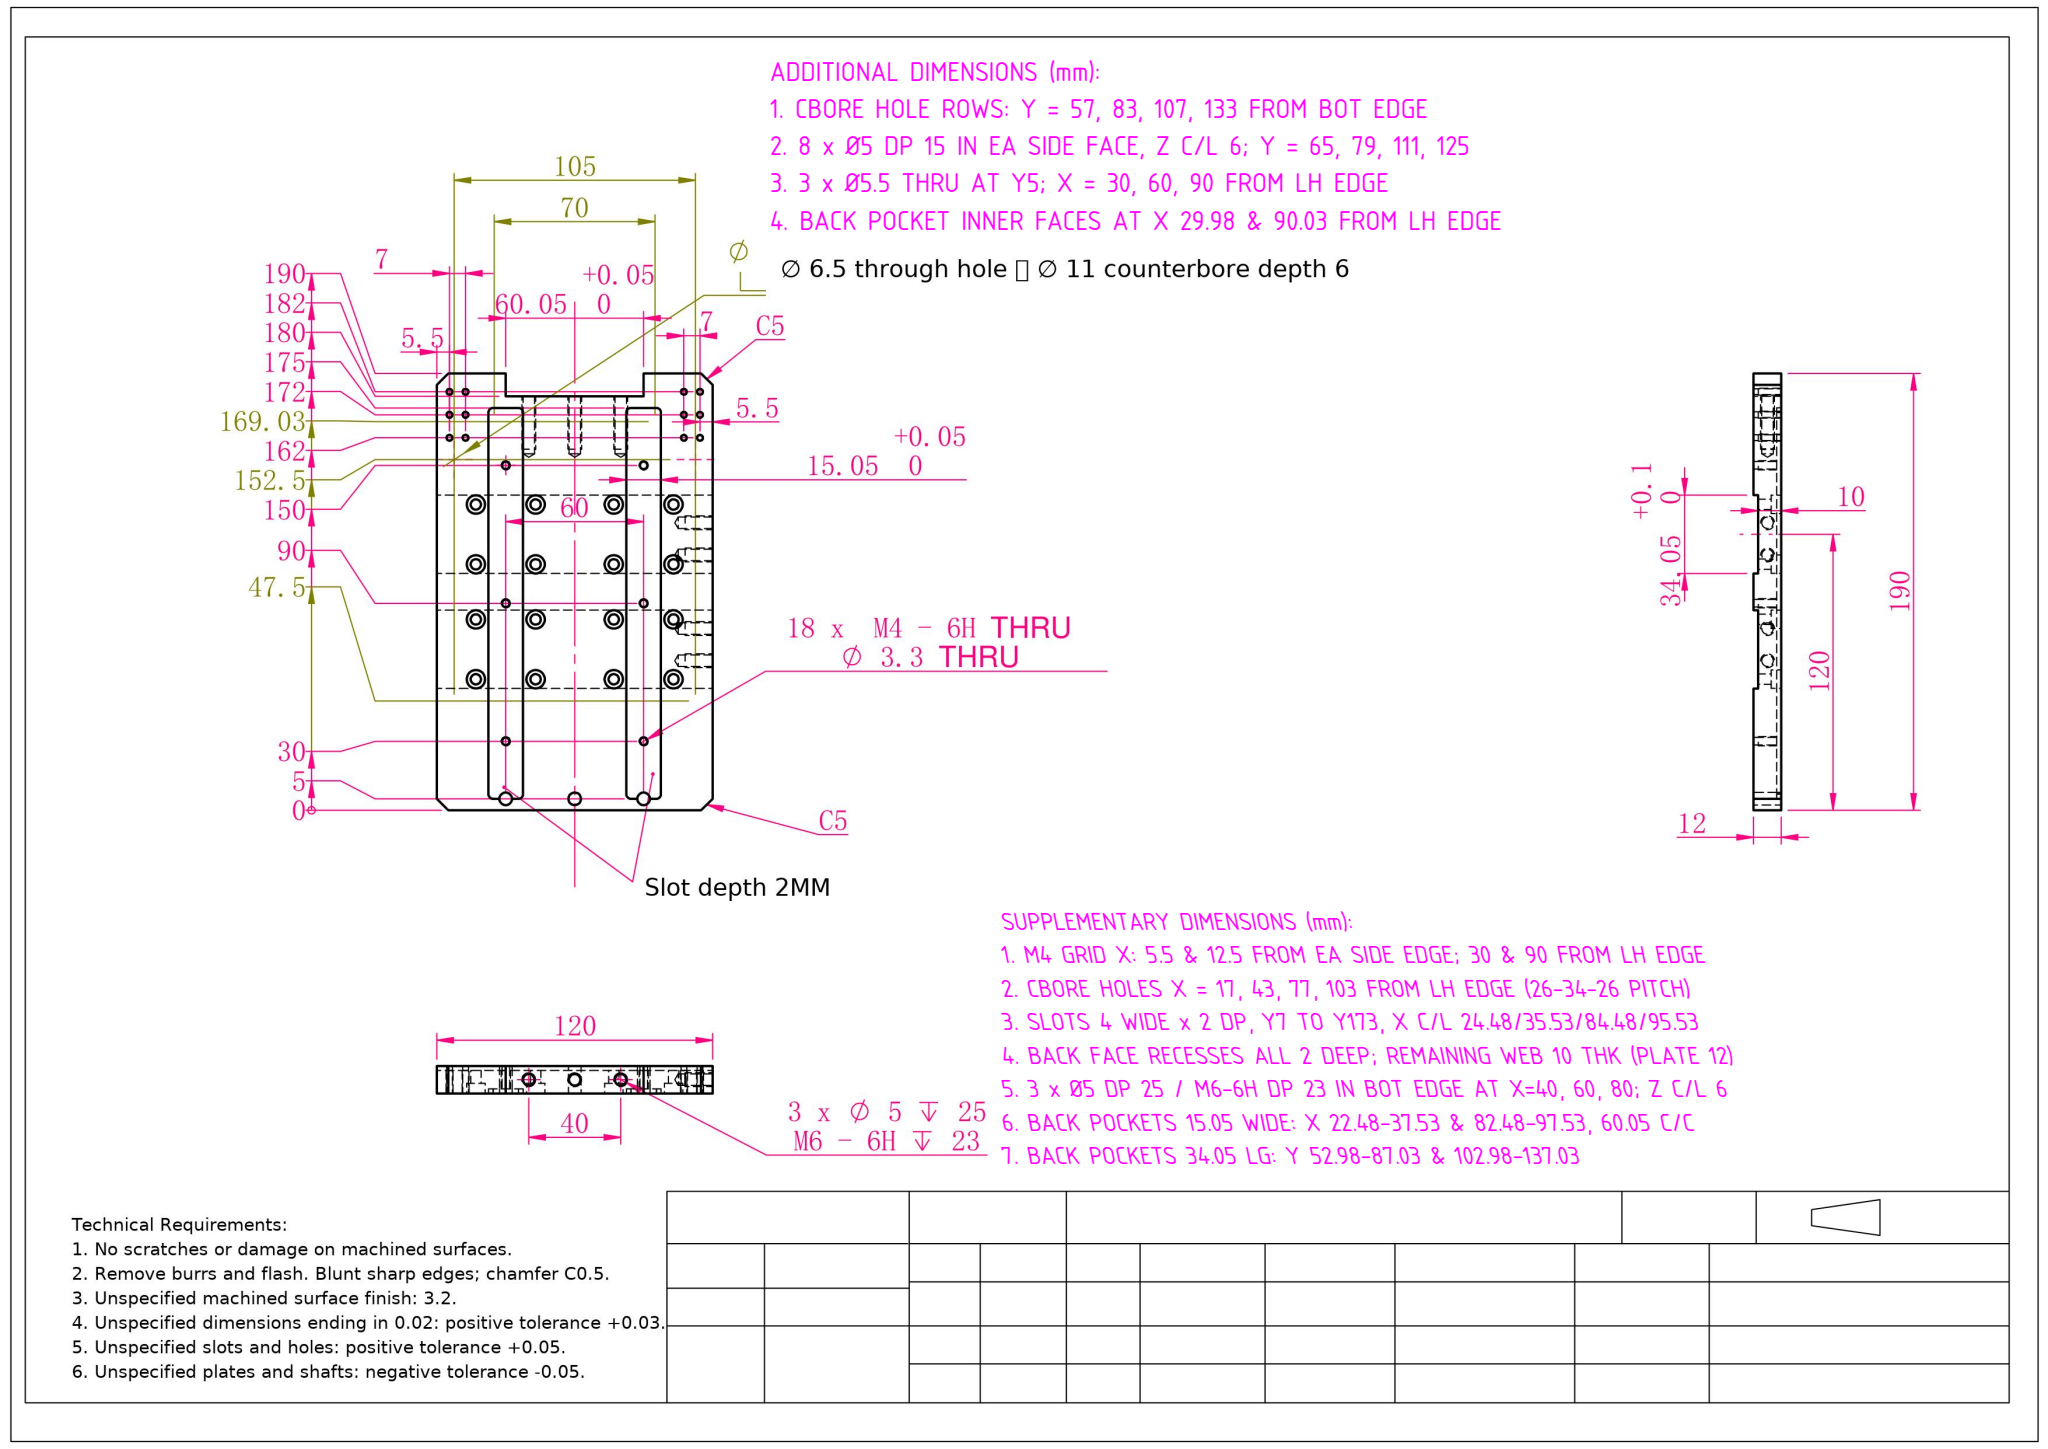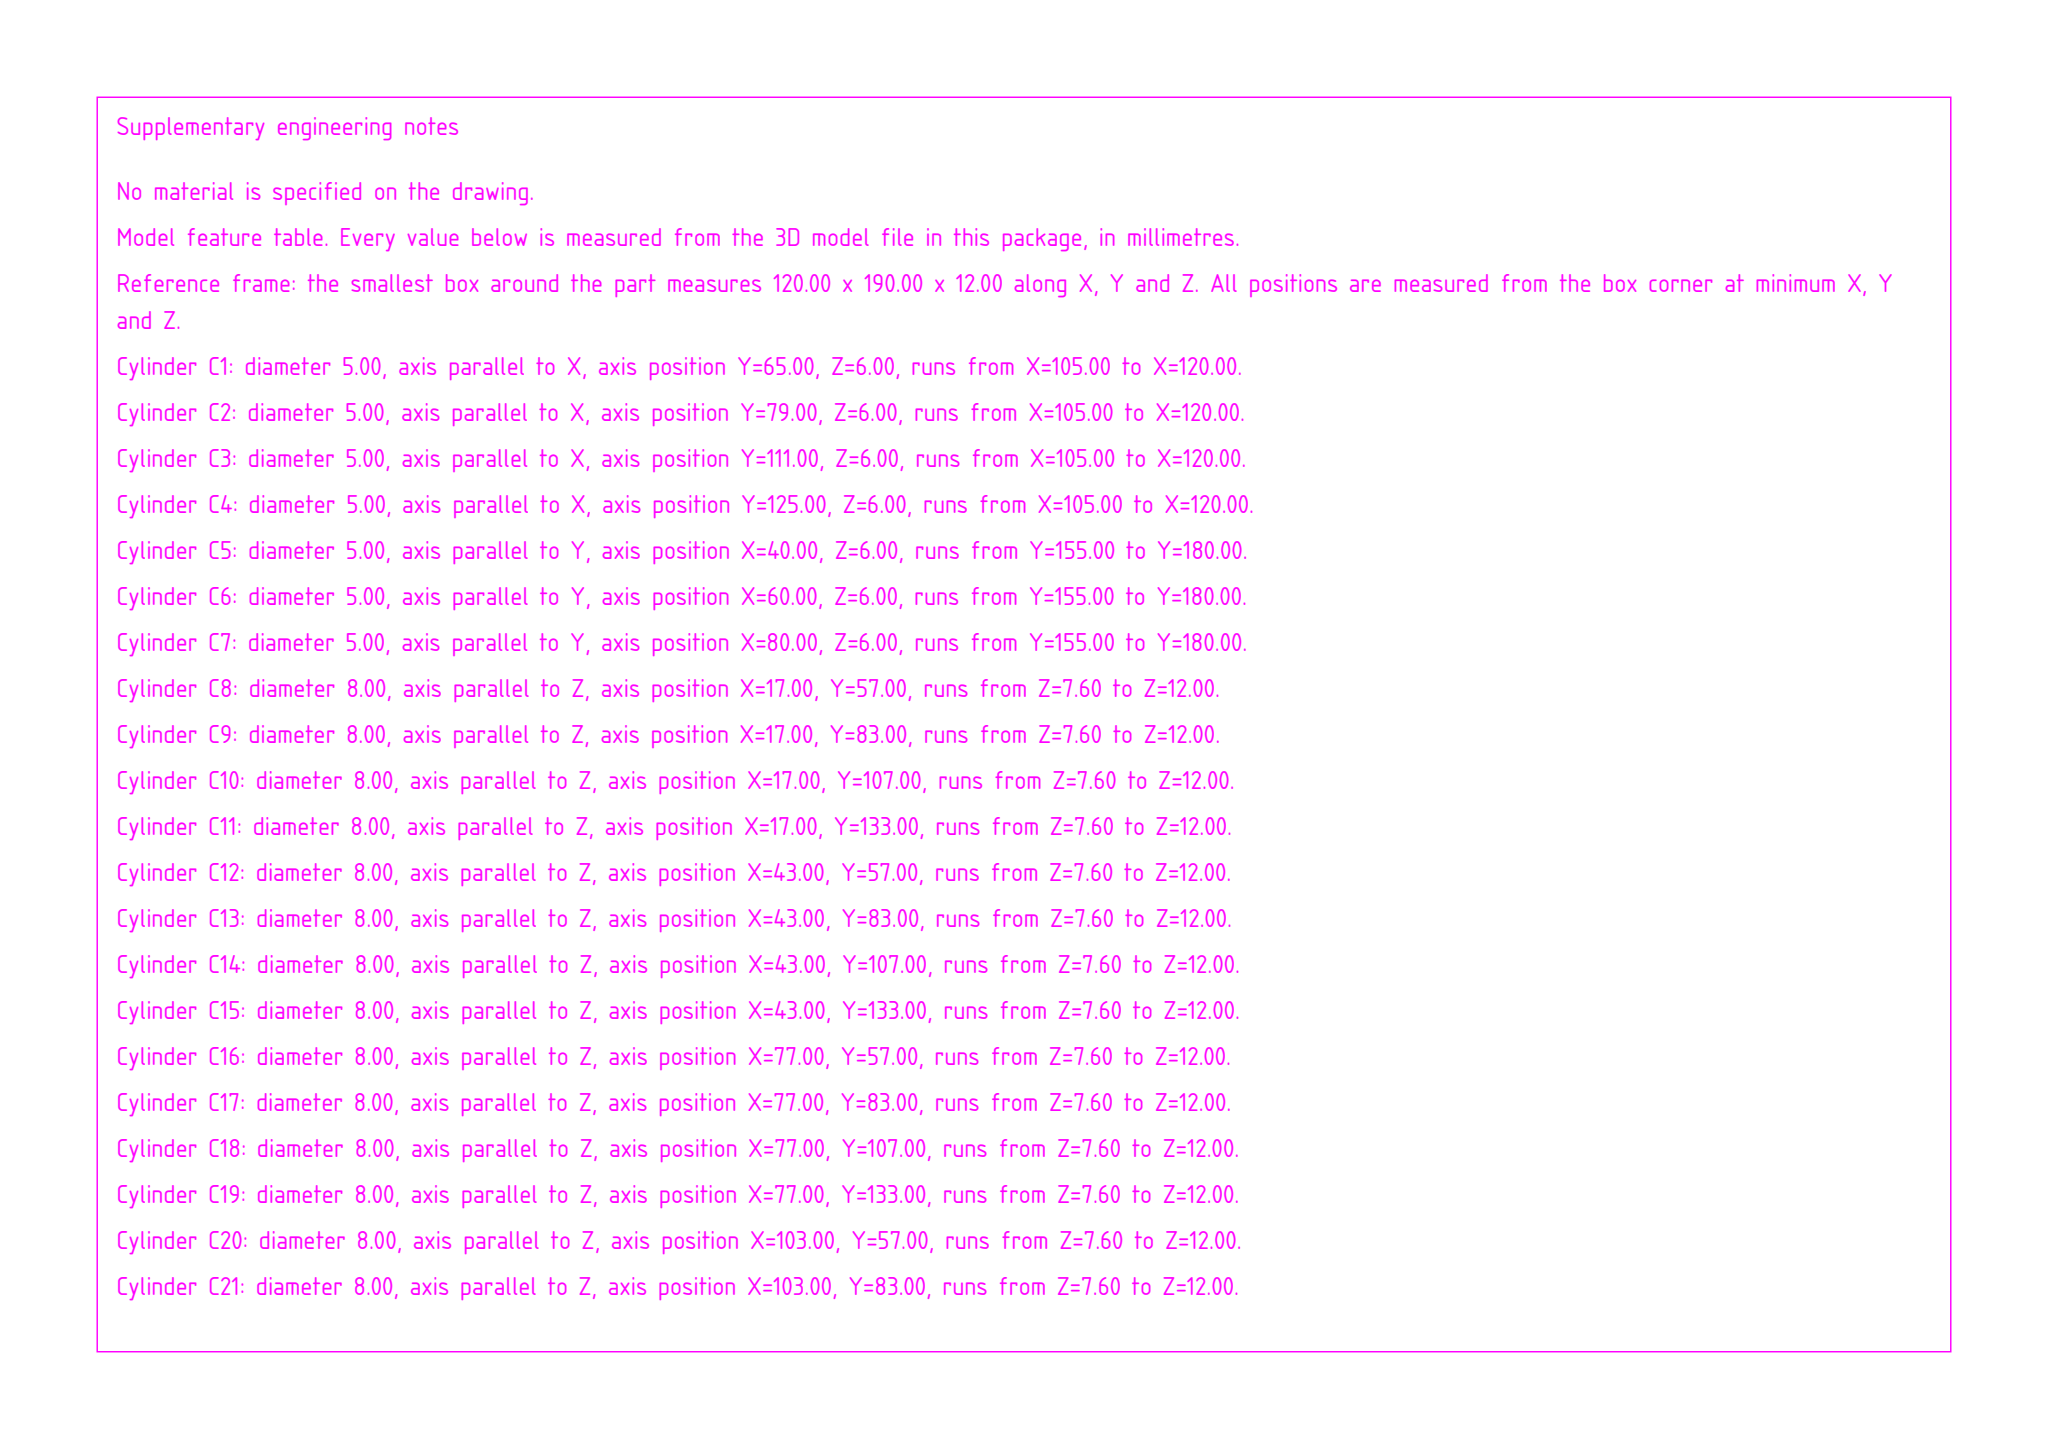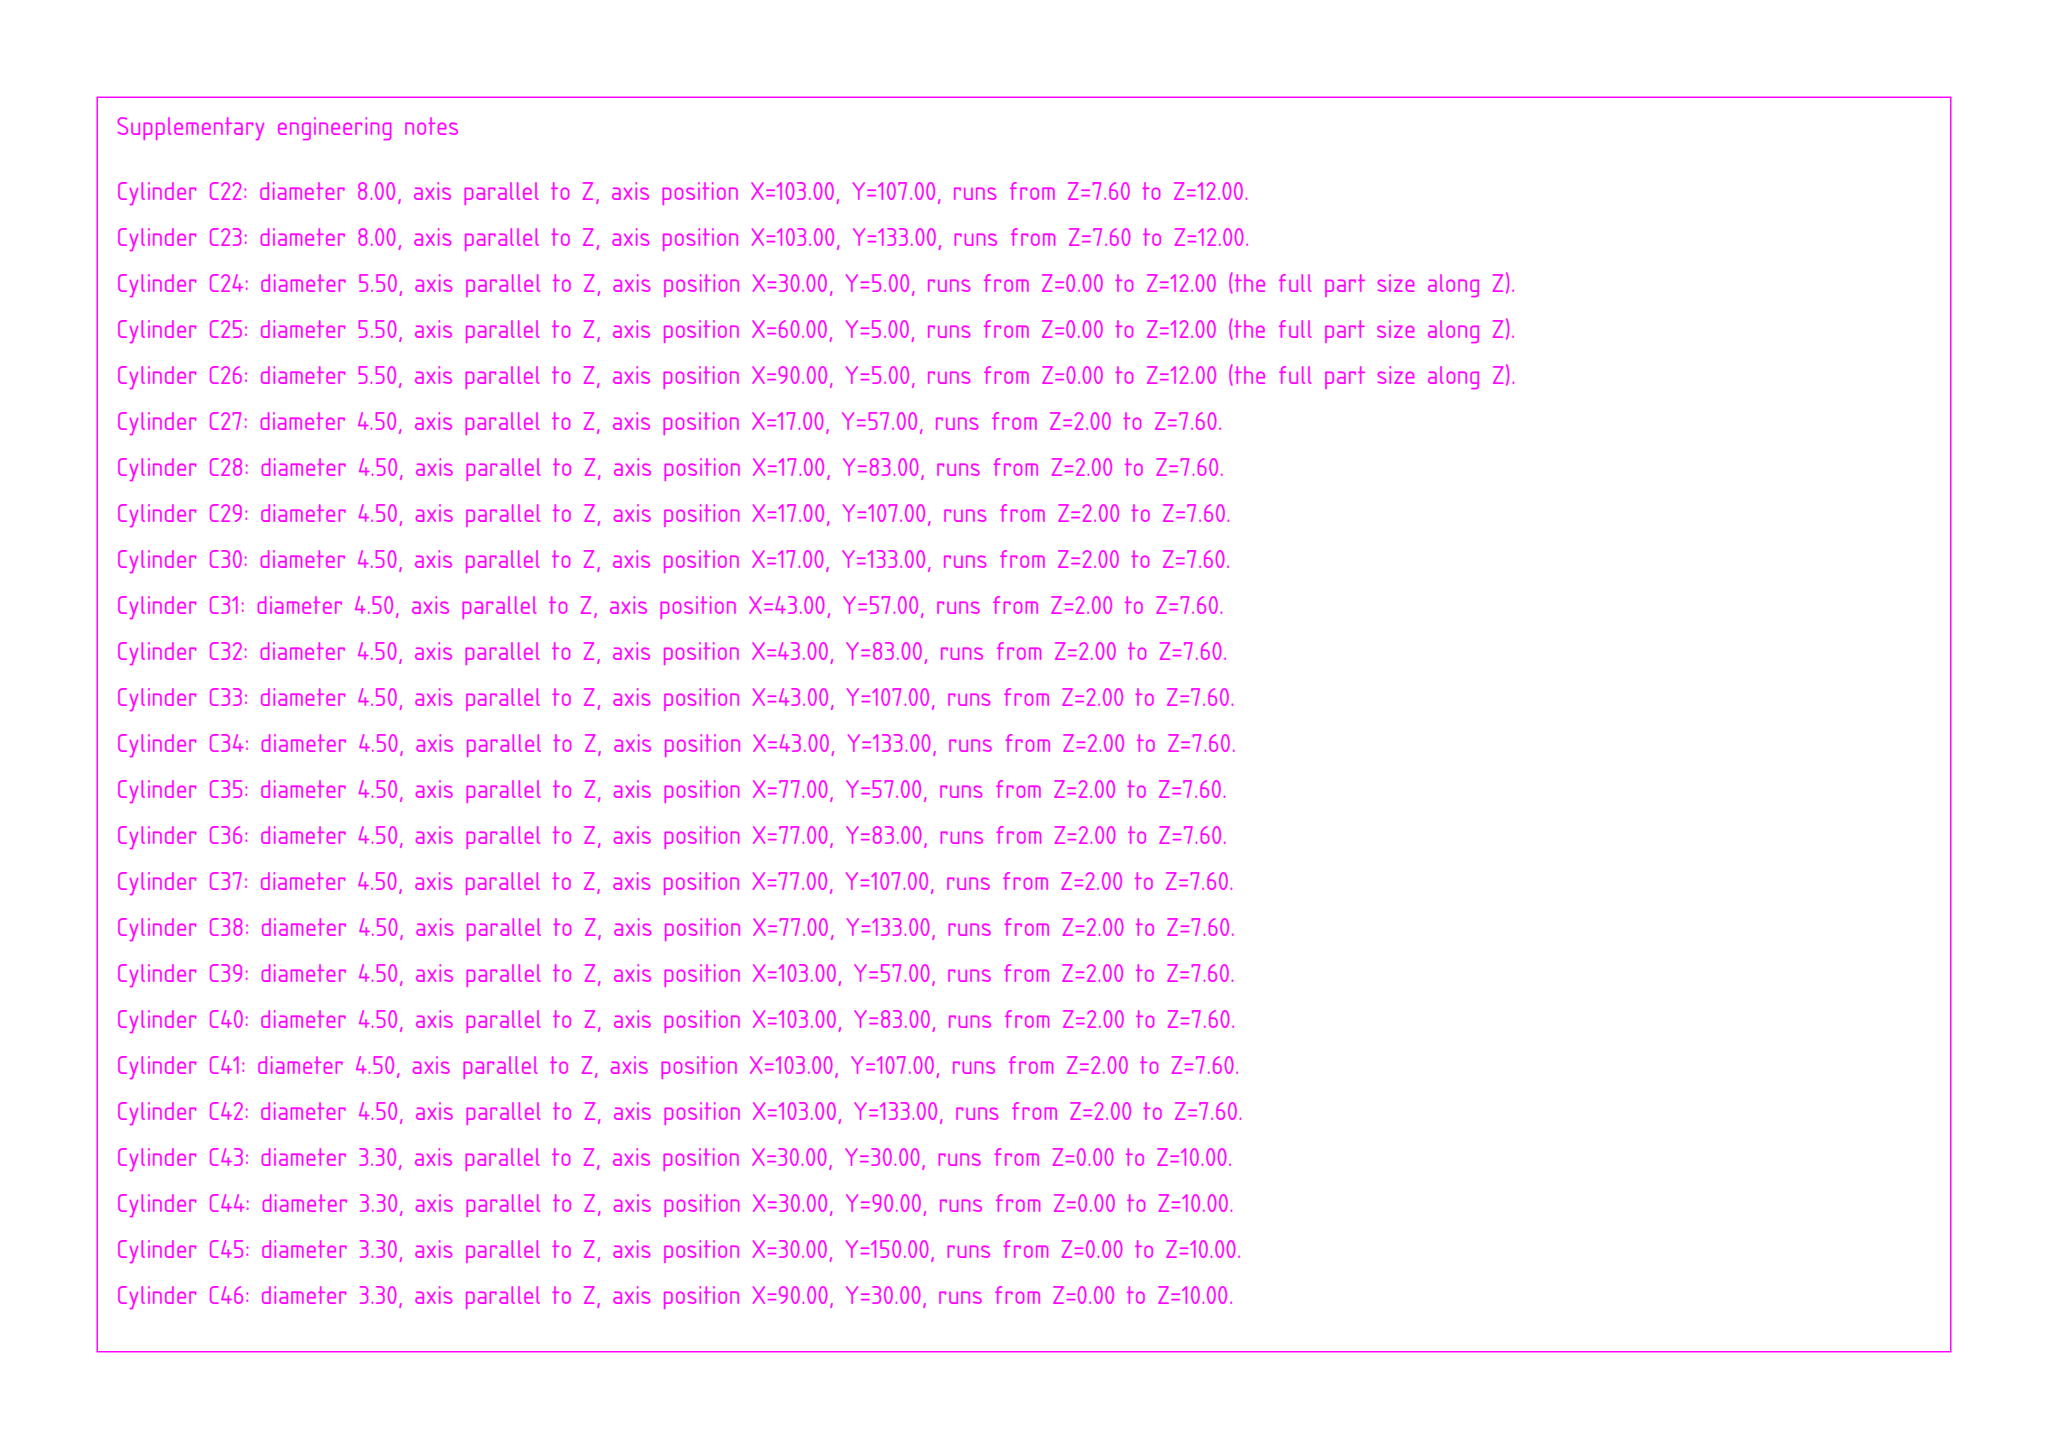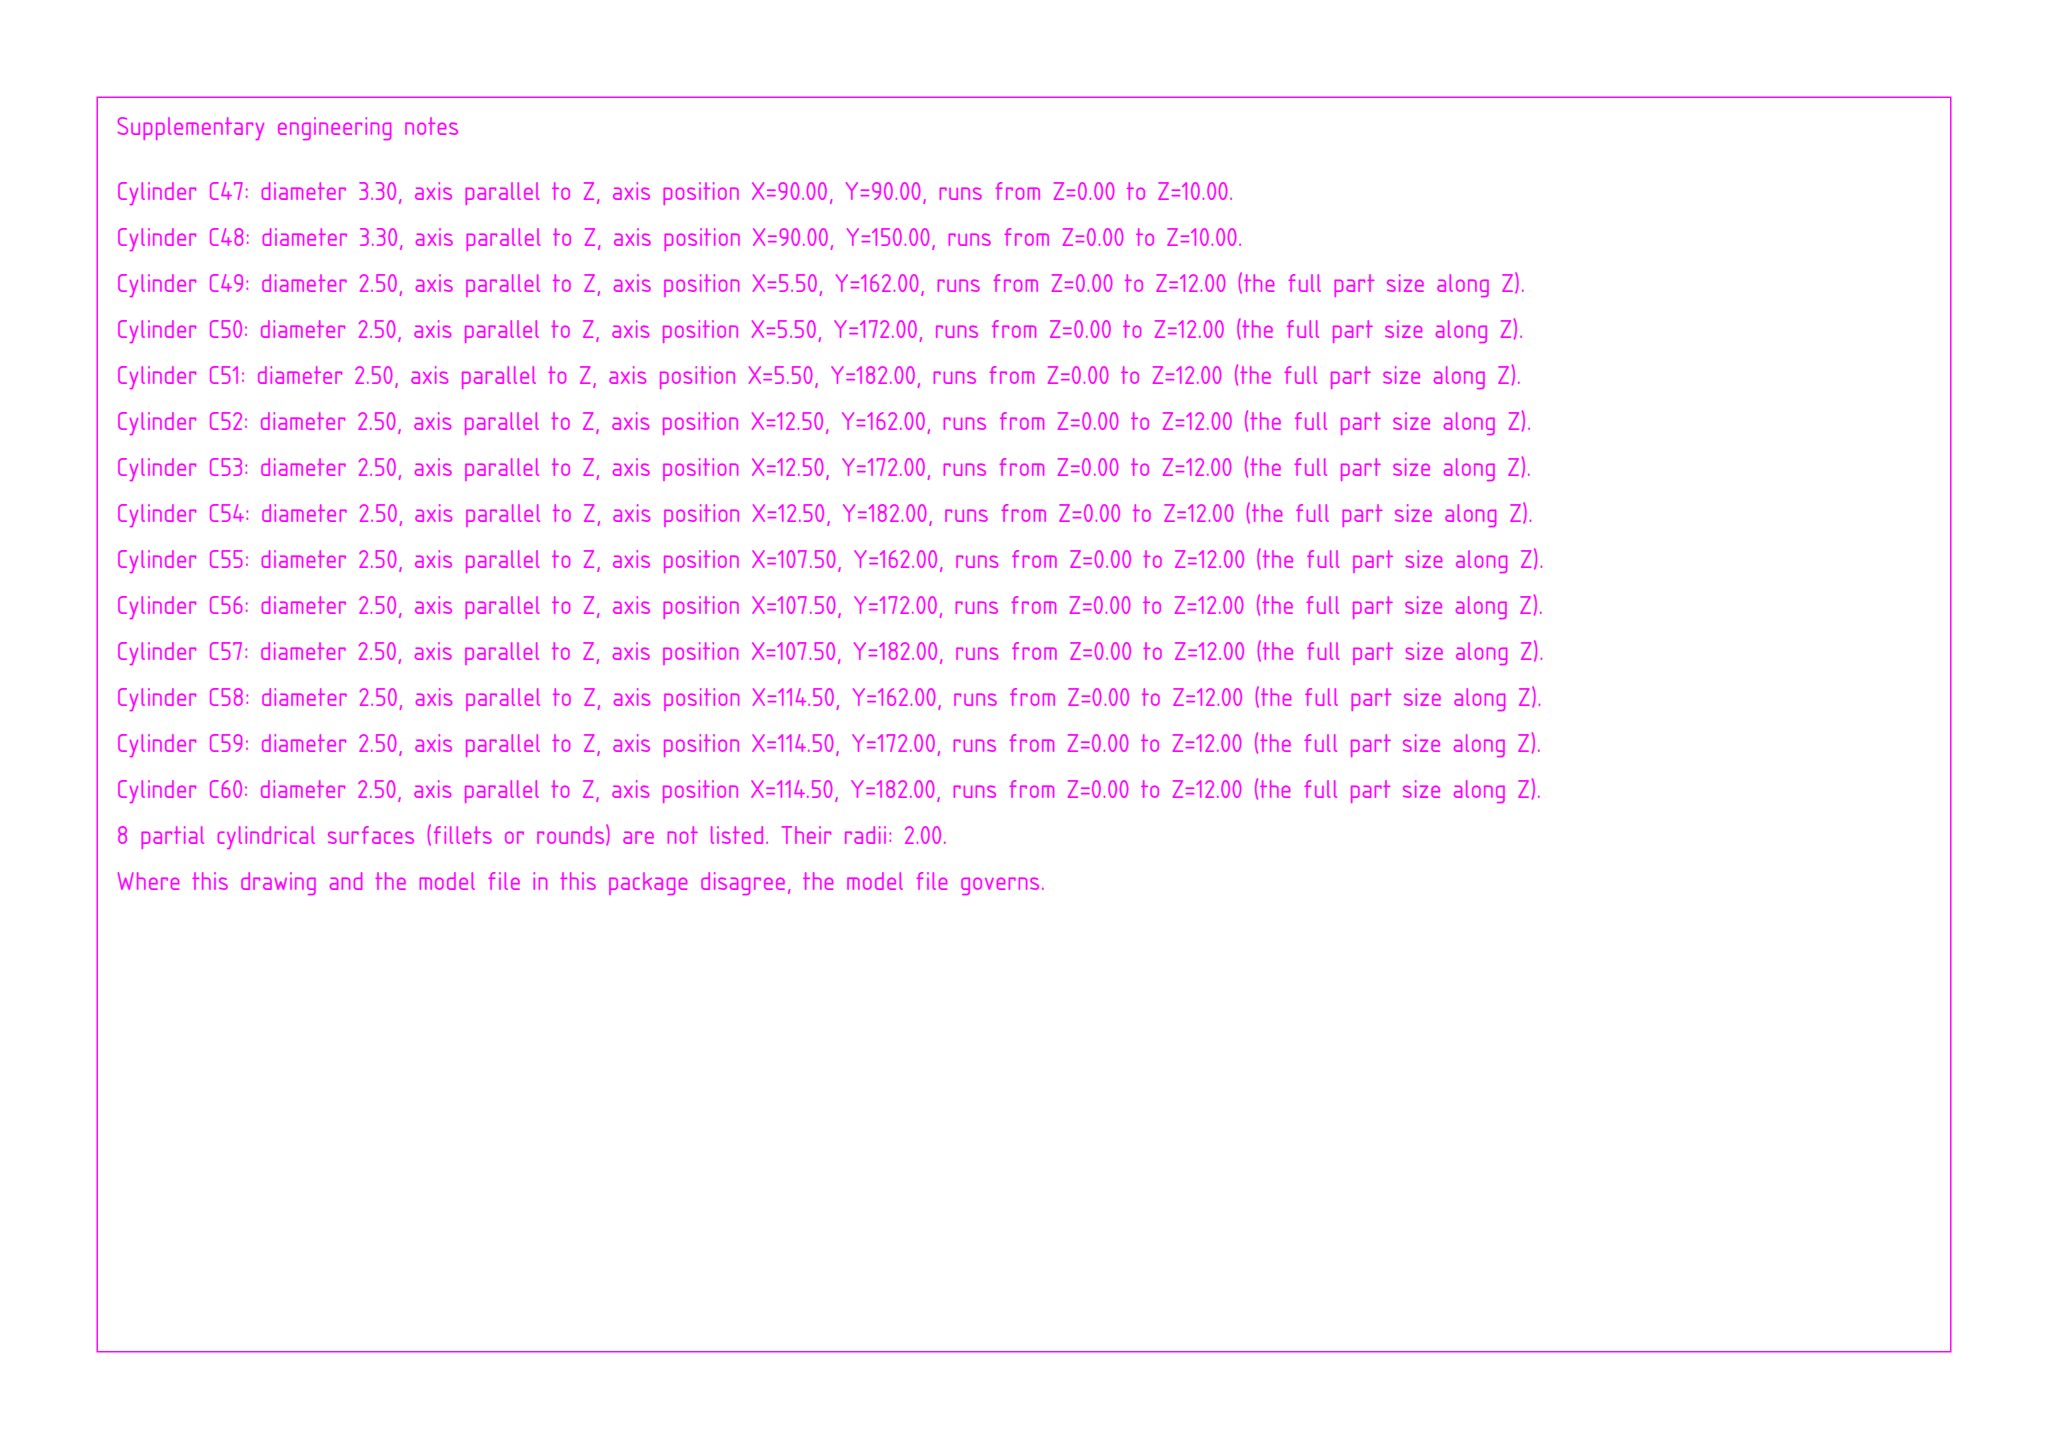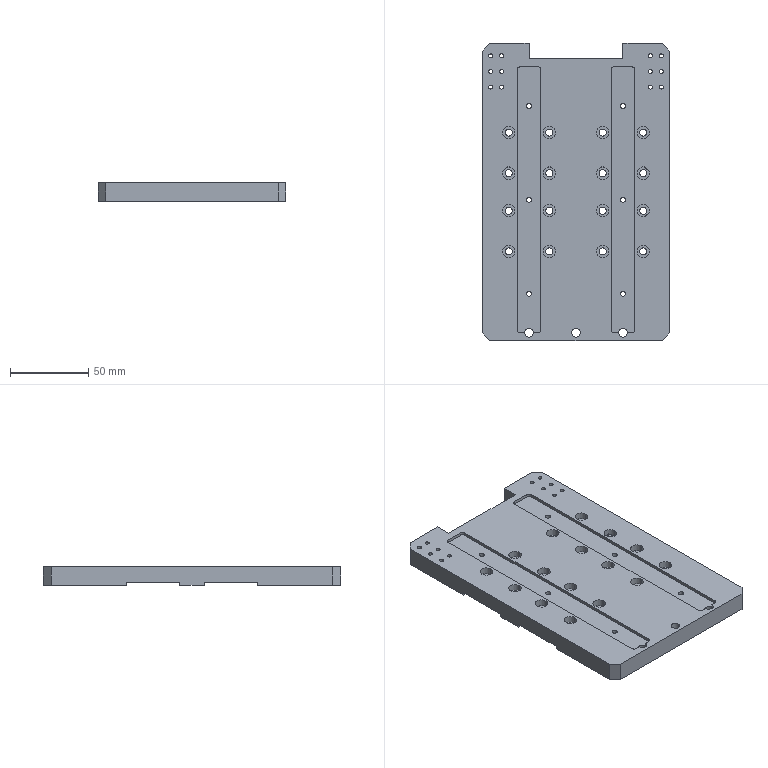Part | SolidWorks | mm | 1 solid | 192 faces | box 120 x 190 x 12 mm | volume 229520 mm3 | cylinder 128 | plane 50 | cone 14 | commonest cylinder face diameters 8 x32 4.5 x32 2.5 x24 5 x14 3.3 x12 4 x8 5.5 x6
build123d program:
from build123d import *

# Parameters (mm, degrees)
SKETCH1_W                                       = 120
SKETCH1_H                                       = 190
BOSS_EXTRUDE1_DEPTH                             = 12
M4_TAPPED_HOLE1_D                               = 3.3
SKETCH13_W                                      = 15.05
SKETCH13_H                                      = 170
CUT_EXTRUDE1_DEPTH                              = 2
SKETCH14_W                                      = 60.05
SKETCH14_H                                      = 10
CUT_EXTRUDE2_DEPTH                              = 114
M6_TAPPED_HOLE1_D                               = 5
M6_TAPPED_HOLE1_DEPTH                           = 25
M6_TAPPED_HOLE1_TIP                             = 1.502
FILLET1_R                                       = 2
M5_CLEARANCE_HOLE1_D                            = 5.5
M3_TAPPED_HOLE1_D                               = 2.5
LPATTERN2_COUNT                                 = 3
LPATTERN2_PITCH                                 = 10
MIRROR1_COPY_1_D                                = 2.5
MIRROR1_COPY_2_D                                = 2.5
SKETCH24_W                                      = 120
SKETCH24_H                                      = 34.05
CUT_EXTRUDE3_DEPTH                              = 2
M4_HEX_SOCKET_HEAD_CAP_SCREW_CBORE1_D           = 4.5
M4_HEX_SOCKET_HEAD_CAP_SCREW_CBORE1_CBORE_D     = 8
M4_HEX_SOCKET_HEAD_CAP_SCREW_CBORE1_CBORE_DEPTH = 4.4
CHAMFER1_SIZE                                   = 5
M6_TAPPED_HOLE2_D                               = 5
M6_TAPPED_HOLE2_DEPTH                           = 15
M6_TAPPED_HOLE2_TIP                             = 1.502
LPATTERN3_COUNT                                 = 2
LPATTERN3_PITCH                                 = 50


with BuildPart() as part:
    # Sketch1 → Boss-Extrude1 (new body)
    with BuildSketch(Plane.XY):
        Rectangle(SKETCH1_W, SKETCH1_H)
    extrude(amount=BOSS_EXTRUDE1_DEPTH)

    # M4 Tapped Hole1 (through all)
    with Locations(Plane.XY.offset(12)):
        with Locations((-30, 55), (30, 55), (-30, -5), (30, -5), (-30, -65), (30, -65), (-30, -125), (30, -125), (-30, -185), (30, -185), (-30, -245), (30, -245), (-30, -305), (30, -305), (-30, -365), (30, -365), (-30, -425), (30, -425)):
            Hole(M4_TAPPED_HOLE1_D / 2)

    # Sketch13 → Cut-Extrude1 (cut)
    with BuildSketch(Plane.XY.offset(12)):
        with Locations((-30, -5)):
            Rectangle(SKETCH13_W, SKETCH13_H)
        with Locations((30, -5)):
            Rectangle(SKETCH13_W, SKETCH13_H)
    extrude(amount=-CUT_EXTRUDE1_DEPTH, mode=Mode.SUBTRACT)

    # Sketch14 → Cut-Extrude2 (cut, through all)
    with BuildSketch(Plane.XY.offset(12)):
        with Locations((0, 90)):
            Rectangle(SKETCH14_W, SKETCH14_H)
    extrude(amount=-CUT_EXTRUDE2_DEPTH, mode=Mode.SUBTRACT)

    # M6 Tapped Hole1
    with Locations(Plane(origin=(0, 85, 0), x_dir=(1, 0, 0), z_dir=(0, 1, 0))):
        with Locations((-20, -6), (20, -6), (0, -6)):
            Hole(M6_TAPPED_HOLE1_D / 2, depth=M6_TAPPED_HOLE1_DEPTH)
            with Locations((0, 0, -(M6_TAPPED_HOLE1_DEPTH + M6_TAPPED_HOLE1_TIP / 2))):  # 118° drill point
                Cone(0, M6_TAPPED_HOLE1_D / 2, M6_TAPPED_HOLE1_TIP, mode=Mode.SUBTRACT)

    # Fillet1
    fillet1_edges = [part.edges().sort_by_distance(p)[0] for p in [
        (-37.525, -90, 11),
        (-37.525, 80, 11),
        (-22.475, 80, 11),
        (-22.475, -90, 11),
        (22.475, 80, 11),
        (37.525, 80, 11),
        (37.525, -90, 11),
        (22.475, -90, 11),
    ]]
    fillet(fillet1_edges, radius=FILLET1_R)

    # M5 Clearance Hole1 (through all)
    with Locations(Plane(origin=(0, 0, 0), x_dir=(-1, 0, 0), z_dir=(0, 0, -1))):
        with Locations((-30, -90), (0, -90), (30, -90)):
            Hole(M5_CLEARANCE_HOLE1_D / 2)

    # M3 Tapped Hole1 (through all)
    with Locations(Plane.XY.offset(12)):
        with Locations((47.5, 67), (54.5, 67)):
            m3_tapped_hole1 = Hole(M3_TAPPED_HOLE1_D / 2)

    # LPattern2: M3 Tapped Hole1 ×3
    with Locations(*[(0, i * LPATTERN2_PITCH, 0) for i in range(1, LPATTERN2_COUNT)]):
        add(m3_tapped_hole1, mode=Mode.SUBTRACT)

    # Mirror1: M3 Tapped Hole1 across plane
    add(m3_tapped_hole1.mirror(Plane(origin=(0, 0, 0), x_dir=(0, 0, 1), z_dir=(1, 0, 0))), mode=Mode.SUBTRACT)

    # Mirror1 copy 1 (through all)
    with Locations(Plane(origin=(0, 10, 12), x_dir=(-1, 0, 0), z_dir=(0, 0, 1))):
        with Locations((47.5, -67), (54.5, -67)):
            Hole(MIRROR1_COPY_1_D / 2)

    # Mirror1 copy 2 (through all)
    with Locations(Plane(origin=(0, 20, 12), x_dir=(-1, 0, 0), z_dir=(0, 0, 1))):
        with Locations((47.5, -67), (54.5, -67)):
            Hole(MIRROR1_COPY_2_D / 2)

    # Sketch24 → Cut-Extrude3 (cut)
    with BuildSketch(Plane(origin=(0, 0, 0), x_dir=(-1, 0, 0), z_dir=(0, 0, -1))):
        with Locations((0, 25)):
            Rectangle(SKETCH24_W, SKETCH24_H)
        with Locations((0, -25)):
            Rectangle(SKETCH24_W, SKETCH24_H)
    extrude(amount=-CUT_EXTRUDE3_DEPTH, mode=Mode.SUBTRACT)

    # M4 Hex Socket Head Cap Screw CBORE1 (through all)
    with Locations(Plane.XY.offset(12)):
        with Locations((17, 38), (43, 38), (-17, 38), (-43, 38), (43, 12), (17, 12), (-43, 12), (-17, 12)):
            m4_hex_socket_head_cap_screw_cbore1 = CounterBoreHole(M4_HEX_SOCKET_HEAD_CAP_SCREW_CBORE1_D / 2, M4_HEX_SOCKET_HEAD_CAP_SCREW_CBORE1_CBORE_D / 2, M4_HEX_SOCKET_HEAD_CAP_SCREW_CBORE1_CBORE_DEPTH)

    # Chamfer1
    chamfer1_edges = [part.edges().sort_by_distance(p)[0] for p in [
        (60, 95, 6),
        (60, -95, 6),
        (-60, -95, 6),
        (-60, 95, 6),
    ]]
    chamfer(chamfer1_edges, length=CHAMFER1_SIZE)

    # M6 Tapped Hole2
    with Locations(Plane(origin=(60, 0, 0), x_dir=(0, 0, -1), z_dir=(1, 0, 0))):
        with Locations((-6, -16), (-6, -30), (-6, 30), (-6, 16)):
            Hole(M6_TAPPED_HOLE2_D / 2, depth=M6_TAPPED_HOLE2_DEPTH)
            with Locations((0, 0, -(M6_TAPPED_HOLE2_DEPTH + M6_TAPPED_HOLE2_TIP / 2))):  # 118° drill point
                Cone(0, M6_TAPPED_HOLE2_D / 2, M6_TAPPED_HOLE2_TIP, mode=Mode.SUBTRACT)

    # LPattern3: M4 Hex Socket Head Cap Screw CBORE1 ×2
    with Locations(*[(0, -i * LPATTERN3_PITCH, 0) for i in range(1, LPATTERN3_COUNT)]):
        add(m4_hex_socket_head_cap_screw_cbore1, mode=Mode.SUBTRACT)


solid = part.part